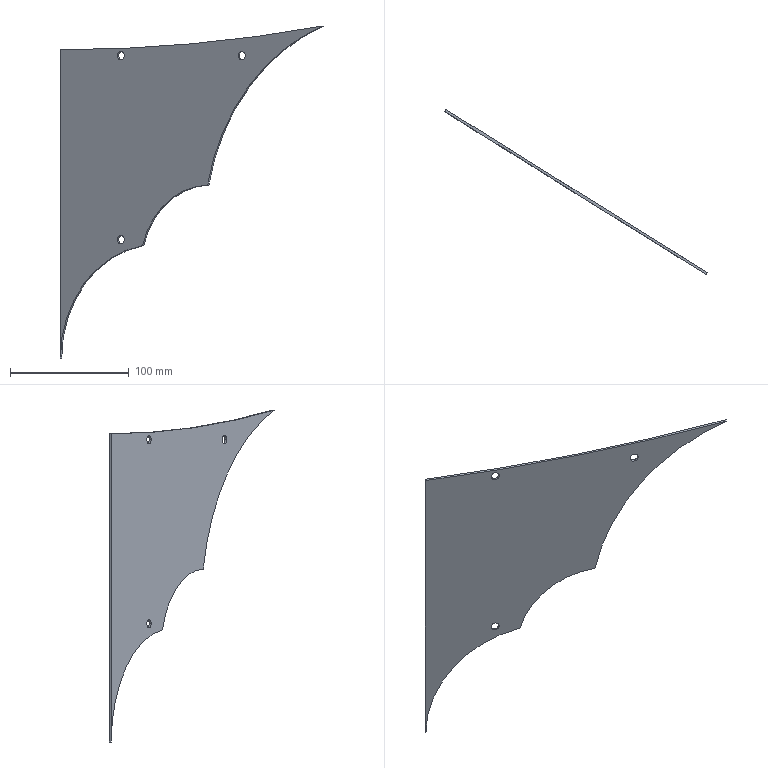Component | SolidWorks | OuterWing-2 | 1 solid | 13 faces | box 221.61 x 139.38 x 279.64 mm | volume 55641 mm3 | cylinder 10 | plane 3 | commonest cylinder face diameters 7 x6 3400 x1 361.12 x1 137.802 x1 191.397 x1
build123d program:
from build123d import *

# Parameters (mm, degrees)
SKETCH1_W           = 260
SKETCH1_H           = 165
BOSS_EXTRUDE1_DEPTH = 2
SKETCH2_R           = 3.5
CUT_EXTRUDE1_DEPTH  = 2
BOSS_EXTRUDE2_DEPTH = 2
CUT_EXTRUDE2_DEPTH  = 2
BOSS_EXTRUDE3_DEPTH = 2


with BuildPart() as part:
    # Sketch1 → Boss-Extrude1 (new body)
    with BuildSketch(Plane.XY):
        with Locations((224.486, -82.5)):
            Rectangle(SKETCH1_W, SKETCH1_H)
    extrude(amount=BOSS_EXTRUDE1_DEPTH)

    # Sketch2 → Cut-Extrude1 (cut)
    with BuildSketch(Plane.XY.offset(2)):
        with Locations((154.486, -160)):
            Circle(SKETCH2_R)
        with Locations((274.486, -160)):
            Circle(SKETCH2_R)
        with Locations((154.486, -5)):
            Circle(SKETCH2_R)
    extrude(amount=-CUT_EXTRUDE1_DEPTH, mode=Mode.SUBTRACT)

    # Sketch3 → Boss-Extrude2 (add)
    with BuildSketch(Plane.XY.offset(2)):
        with BuildLine():
            Line((354.486, -165), (354.486, -185))
            ThreePointArc((354.486, -185), (224.87, -170.007), (94.486, -165))
            Line((94.486, -165), (354.486, -165))
        make_face()
    extrude(amount=-BOSS_EXTRUDE2_DEPTH)

    # Sketch4 → Cut-Extrude2 (cut)
    with BuildSketch(Plane.XY.offset(2)):
        with BuildLine():
            Line((175.984, 0), (354.486, 0))
            Line((354.486, 0), (354.486, -185))
            ThreePointArc((354.486, -185), (280.155, -132.818), (240.63, -51.051))
            ThreePointArc((240.63, -51.051), (199.838, -36.25), (175.984, 0))
        make_face()
    extrude(amount=-CUT_EXTRUDE2_DEPTH, mode=Mode.SUBTRACT)

    # Sketch5 → Boss-Extrude3 (add)
    with BuildSketch(Plane(origin=(0, 0, 0), x_dir=(-1, 0, 0), z_dir=(0, 0, -1))):
        with BuildLine():
            Line((-94.486, 0), (-94.486, 94.639))
            ThreePointArc((-94.486, 94.639), (-117.668, 32.192), (-175.984, 0))
            Line((-175.984, 0), (-94.486, 0))
        make_face()
    extrude(amount=-BOSS_EXTRUDE3_DEPTH)


solid = part.part

# Placed as in the assembly
solid = solid.moved(Location((95.28, 103.927, -37.818), (-90, 31.974, 0)))
STEP:
#1=COLOUR_RGB('',0.7922,0.8196,0.9333);
#2=FILL_AREA_STYLE_COLOUR('',#1);
#3=FILL_AREA_STYLE('',(#2));
#4=SURFACE_STYLE_FILL_AREA(#3);
#5=SURFACE_SIDE_STYLE('',(#4));
#6=SURFACE_STYLE_USAGE(.BOTH.,#5);
#7=PRESENTATION_STYLE_ASSIGNMENT((#6));
#8=CARTESIAN_POINT('',(8.794,0.9439,-1.292));
#9=VERTEX_POINT('',#8);
#10=CARTESIAN_POINT('',(9.027,0.7979,-1.292));
#11=VERTEX_POINT('',#10);
#12=CARTESIAN_POINT('',(8.911,0.8709,-1.292));
#13=DIRECTION('',(0.5295,0.8483,-0.));
#14=DIRECTION('',(0.8483,-0.5295,-0.));
#15=AXIS2_PLACEMENT_3D('',#12,#13,#14);
#16=CIRCLE('',#15,0.1378);
#17=EDGE_CURVE('',#9,#11,#16,.T.);
#18=ORIENTED_EDGE('',*,*,#17,.F.);
#19=CARTESIAN_POINT('',(8.835,1.011,-1.292));
#20=VERTEX_POINT('',#19);
#21=CARTESIAN_POINT('',(8.794,0.9439,-1.292));
#22=DIRECTION('',(0.5295,0.8483,-0.));
#23=VECTOR('',#22,39.37);
#24=LINE('',#21,#23);
#25=EDGE_CURVE('',#9,#20,#24,.T.);
#26=ORIENTED_EDGE('',*,*,#25,.T.);
#27=CARTESIAN_POINT('',(9.069,0.8647,-1.292));
#28=VERTEX_POINT('',#27);
#29=CARTESIAN_POINT('',(8.952,0.9377,-1.292));
#30=DIRECTION('',(0.5295,0.8483,-0.));
#31=DIRECTION('',(0.8483,-0.5295,-0.));
#32=AXIS2_PLACEMENT_3D('',#29,#30,#31);
#33=CIRCLE('',#32,0.1378);
#34=EDGE_CURVE('',#20,#28,#33,.T.);
#35=ORIENTED_EDGE('',*,*,#34,.T.);
#36=CARTESIAN_POINT('',(9.027,0.7979,-1.292));
#37=DIRECTION('',(0.5295,0.8483,-0.));
#38=VECTOR('',#37,39.37);
#39=LINE('',#36,#38);
#40=EDGE_CURVE('',#11,#28,#39,.T.);
#41=ORIENTED_EDGE('',*,*,#40,.F.);
#42=EDGE_LOOP('',(#18,#26,#35,#41));
#43=FACE_OUTER_BOUND('',#42,.T.);
#44=CARTESIAN_POINT('',(8.911,0.8709,-1.292));
#45=DIRECTION('',(0.5295,0.8483,-0.));
#46=DIRECTION('',(0.8483,-0.5295,-0.));
#47=AXIS2_PLACEMENT_3D('',#44,#45,#46);
#48=CYLINDRICAL_SURFACE('',#47,0.1378);
#49=ADVANCED_FACE('',(#43),#48,.F.);
#50=CARTESIAN_POINT('',(12.801,-1.558,4.81));
#51=VERTEX_POINT('',#50);
#52=CARTESIAN_POINT('',(13.035,-1.704,4.81));
#53=VERTEX_POINT('',#52);
#54=CARTESIAN_POINT('',(12.918,-1.631,4.81));
#55=DIRECTION('',(0.5295,0.8483,-0.));
#56=DIRECTION('',(0.8483,-0.5295,-0.));
#57=AXIS2_PLACEMENT_3D('',#54,#55,#56);
#58=CIRCLE('',#57,0.1378);
#59=EDGE_CURVE('',#51,#53,#58,.T.);
#60=ORIENTED_EDGE('',*,*,#59,.F.);
#61=CARTESIAN_POINT('',(12.843,-1.491,4.81));
#62=VERTEX_POINT('',#61);
#63=CARTESIAN_POINT('',(12.801,-1.558,4.81));
#64=DIRECTION('',(0.5295,0.8483,-0.));
#65=VECTOR('',#64,39.37);
#66=LINE('',#63,#65);
#67=EDGE_CURVE('',#51,#62,#66,.T.);
#68=ORIENTED_EDGE('',*,*,#67,.T.);
#69=CARTESIAN_POINT('',(13.077,-1.637,4.81));
#70=VERTEX_POINT('',#69);
#71=CARTESIAN_POINT('',(12.96,-1.564,4.81));
#72=DIRECTION('',(0.5295,0.8483,-0.));
#73=DIRECTION('',(0.8483,-0.5295,-0.));
#74=AXIS2_PLACEMENT_3D('',#71,#72,#73);
#75=CIRCLE('',#74,0.1378);
#76=EDGE_CURVE('',#62,#70,#75,.T.);
#77=ORIENTED_EDGE('',*,*,#76,.T.);
#78=CARTESIAN_POINT('',(13.035,-1.704,4.81));
#79=DIRECTION('',(0.5295,0.8483,-0.));
#80=VECTOR('',#79,39.37);
#81=LINE('',#78,#80);
#82=EDGE_CURVE('',#53,#70,#81,.T.);
#83=ORIENTED_EDGE('',*,*,#82,.F.);
#84=EDGE_LOOP('',(#60,#68,#77,#83));
#85=FACE_OUTER_BOUND('',#84,.T.);
#86=CARTESIAN_POINT('',(12.918,-1.631,4.81));
#87=DIRECTION('',(0.5295,0.8483,-0.));
#88=DIRECTION('',(0.8483,-0.5295,-0.));
#89=AXIS2_PLACEMENT_3D('',#86,#87,#88);
#90=CYLINDRICAL_SURFACE('',#89,0.1378);
#91=ADVANCED_FACE('',(#85),#90,.F.);
#92=CARTESIAN_POINT('',(8.794,0.9439,4.81));
#93=VERTEX_POINT('',#92);
#94=CARTESIAN_POINT('',(9.027,0.7979,4.81));
#95=VERTEX_POINT('',#94);
#96=CARTESIAN_POINT('',(8.911,0.8709,4.81));
#97=DIRECTION('',(0.5295,0.8483,-0.));
#98=DIRECTION('',(0.8483,-0.5295,-0.));
#99=AXIS2_PLACEMENT_3D('',#96,#97,#98);
#100=CIRCLE('',#99,0.1378);
#101=EDGE_CURVE('',#93,#95,#100,.T.);
#102=ORIENTED_EDGE('',*,*,#101,.F.);
#103=CARTESIAN_POINT('',(8.835,1.011,4.81));
#104=VERTEX_POINT('',#103);
#105=CARTESIAN_POINT('',(8.794,0.9439,4.81));
#106=DIRECTION('',(0.5295,0.8483,-0.));
#107=VECTOR('',#106,39.37);
#108=LINE('',#105,#107);
#109=EDGE_CURVE('',#93,#104,#108,.T.);
#110=ORIENTED_EDGE('',*,*,#109,.T.);
#111=CARTESIAN_POINT('',(9.069,0.8647,4.81));
#112=VERTEX_POINT('',#111);
#113=CARTESIAN_POINT('',(8.952,0.9377,4.81));
#114=DIRECTION('',(0.5295,0.8483,-0.));
#115=DIRECTION('',(0.8483,-0.5295,-0.));
#116=AXIS2_PLACEMENT_3D('',#113,#114,#115);
#117=CIRCLE('',#116,0.1378);
#118=EDGE_CURVE('',#104,#112,#117,.T.);
#119=ORIENTED_EDGE('',*,*,#118,.T.);
#120=CARTESIAN_POINT('',(9.027,0.7979,4.81));
#121=DIRECTION('',(0.5295,0.8483,-0.));
#122=VECTOR('',#121,39.37);
#123=LINE('',#120,#122);
#124=EDGE_CURVE('',#95,#112,#123,.T.);
#125=ORIENTED_EDGE('',*,*,#124,.F.);
#126=EDGE_LOOP('',(#102,#110,#119,#125));
#127=FACE_OUTER_BOUND('',#126,.T.);
#128=CARTESIAN_POINT('',(8.911,0.8709,4.81));
#129=DIRECTION('',(0.5295,0.8483,-0.));
#130=DIRECTION('',(0.8483,-0.5295,-0.));
#131=AXIS2_PLACEMENT_3D('',#128,#129,#130);
#132=CYLINDRICAL_SURFACE('',#131,0.1378);
#133=ADVANCED_FACE('',(#127),#132,.F.);
#134=CARTESIAN_POINT('',(6.907,2.122,-5.215));
#135=VERTEX_POINT('',#134);
#136=CARTESIAN_POINT('',(6.907,2.122,5.007));
#137=VERTEX_POINT('',#136);
#138=CARTESIAN_POINT('',(6.907,2.122,-1.489));
#139=DIRECTION('',(0.,-0.,1.));
#140=VECTOR('',#139,39.37);
#141=LINE('',#138,#140);
#142=EDGE_CURVE('',#135,#137,#141,.T.);
#143=ORIENTED_EDGE('',*,*,#142,.T.);
#144=CARTESIAN_POINT('',(6.948,2.189,5.007));
#145=VERTEX_POINT('',#144);
#146=CARTESIAN_POINT('',(6.948,2.189,5.007));
#147=DIRECTION('',(-0.5295,-0.8483,0.));
#148=VECTOR('',#147,39.37);
#149=LINE('',#146,#148);
#150=EDGE_CURVE('',#145,#137,#149,.T.);
#151=ORIENTED_EDGE('',*,*,#150,.F.);
#152=CARTESIAN_POINT('',(6.948,2.189,-5.215));
#153=VERTEX_POINT('',#152);
#154=CARTESIAN_POINT('',(6.948,2.189,-1.489));
#155=DIRECTION('',(0.,-0.,1.));
#156=VECTOR('',#155,39.37);
#157=LINE('',#154,#156);
#158=EDGE_CURVE('',#153,#145,#157,.T.);
#159=ORIENTED_EDGE('',*,*,#158,.F.);
#160=CARTESIAN_POINT('',(6.948,2.189,-5.215));
#161=DIRECTION('',(-0.5295,-0.8483,0.));
#162=VECTOR('',#161,39.37);
#163=LINE('',#160,#162);
#164=EDGE_CURVE('',#153,#135,#163,.T.);
#165=ORIENTED_EDGE('',*,*,#164,.T.);
#166=EDGE_LOOP('',(#143,#151,#159,#165));
#167=FACE_OUTER_BOUND('',#166,.T.);
#168=CARTESIAN_POINT('',(6.948,2.189,-1.489));
#169=DIRECTION('',(0.8483,-0.5295,-0.));
#170=DIRECTION('',(-0.5295,-0.8483,0.));
#171=AXIS2_PLACEMENT_3D('',#168,#169,#170);
#172=PLANE('',#171);
#173=ADVANCED_FACE('',(#167),#172,.F.);
#174=CARTESIAN_POINT('',(11.829,-0.8582,0.521));
#175=VERTEX_POINT('',#174);
#176=CARTESIAN_POINT('',(15.632,-3.232,5.795));
#177=VERTEX_POINT('',#176);
#178=CARTESIAN_POINT('',(17.744,-4.55,-0.8637));
#179=DIRECTION('',(0.5295,0.8483,-0.));
#180=DIRECTION('',(-0.8483,0.5295,0.));
#181=AXIS2_PLACEMENT_3D('',#178,#179,#180);
#182=CIRCLE('',#181,7.109);
#183=EDGE_CURVE('',#175,#177,#182,.T.);
#184=ORIENTED_EDGE('',*,*,#183,.F.);
#185=CARTESIAN_POINT('',(9.67,0.4895,-1.489));
#186=VERTEX_POINT('',#185);
#187=CARTESIAN_POINT('',(11.893,-0.898,-2.191));
#188=DIRECTION('',(0.5295,0.8483,-0.));
#189=DIRECTION('',(-0.8483,0.5295,0.));
#190=AXIS2_PLACEMENT_3D('',#187,#188,#189);
#191=CIRCLE('',#190,2.713);
#192=EDGE_CURVE('',#186,#175,#191,.T.);
#193=ORIENTED_EDGE('',*,*,#192,.F.);
#194=CARTESIAN_POINT('',(10.144,0.1935,-5.215));
#195=DIRECTION('',(0.5295,0.8483,-0.));
#196=DIRECTION('',(0.8483,-0.5295,-0.));
#197=AXIS2_PLACEMENT_3D('',#194,#195,#196);
#198=CIRCLE('',#197,3.768);
#199=EDGE_CURVE('',#153,#186,#198,.T.);
#200=ORIENTED_EDGE('',*,*,#199,.F.);
#201=ORIENTED_EDGE('',*,*,#158,.T.);
#202=CARTESIAN_POINT('',(6.948,2.189,71.936));
#203=DIRECTION('',(-0.5295,-0.8483,0.));
#204=DIRECTION('',(-0.8483,0.5295,0.));
#205=AXIS2_PLACEMENT_3D('',#202,#203,#204);
#206=CIRCLE('',#205,66.929);
#207=EDGE_CURVE('',#145,#177,#206,.T.);
#208=ORIENTED_EDGE('',*,*,#207,.T.);
#209=EDGE_LOOP('',(#184,#193,#200,#201,#208));
#210=FACE_OUTER_BOUND('',#209,.T.);
#211=CARTESIAN_POINT('',(8.952,0.9377,-1.292));
#212=DIRECTION('',(0.5295,0.8483,-0.));
#213=DIRECTION('',(0.8483,-0.5295,-0.));
#214=AXIS2_PLACEMENT_3D('',#211,#212,#213);
#215=CIRCLE('',#214,0.1378);
#216=EDGE_CURVE('',#28,#20,#215,.T.);
#217=ORIENTED_EDGE('',*,*,#216,.F.);
#218=ORIENTED_EDGE('',*,*,#34,.F.);
#219=EDGE_LOOP('',(#217,#218));
#220=FACE_BOUND('',#219,.T.);
#221=CARTESIAN_POINT('',(12.96,-1.564,4.81));
#222=DIRECTION('',(0.5295,0.8483,-0.));
#223=DIRECTION('',(0.8483,-0.5295,-0.));
#224=AXIS2_PLACEMENT_3D('',#221,#222,#223);
#225=CIRCLE('',#224,0.1378);
#226=EDGE_CURVE('',#70,#62,#225,.T.);
#227=ORIENTED_EDGE('',*,*,#226,.F.);
#228=ORIENTED_EDGE('',*,*,#76,.F.);
#229=EDGE_LOOP('',(#227,#228));
#230=FACE_BOUND('',#229,.T.);
#231=CARTESIAN_POINT('',(8.952,0.9377,4.81));
#232=DIRECTION('',(0.5295,0.8483,-0.));
#233=DIRECTION('',(0.8483,-0.5295,-0.));
#234=AXIS2_PLACEMENT_3D('',#231,#232,#233);
#235=CIRCLE('',#234,0.1378);
#236=EDGE_CURVE('',#112,#104,#235,.T.);
#237=ORIENTED_EDGE('',*,*,#236,.F.);
#238=ORIENTED_EDGE('',*,*,#118,.F.);
#239=EDGE_LOOP('',(#237,#238));
#240=FACE_BOUND('',#239,.T.);
#241=CARTESIAN_POINT('',(3.793,4.158,-1.489));
#242=DIRECTION('',(0.5295,0.8483,-0.));
#243=DIRECTION('',(0.8483,-0.5295,-0.));
#244=AXIS2_PLACEMENT_3D('',#241,#242,#243);
#245=PLANE('',#244);
#246=ADVANCED_FACE('',(#210,#220,#230,#240),#245,.T.);
#247=CARTESIAN_POINT('',(8.911,0.8709,-1.292));
#248=DIRECTION('',(0.5295,0.8483,-0.));
#249=DIRECTION('',(0.8483,-0.5295,-0.));
#250=AXIS2_PLACEMENT_3D('',#247,#248,#249);
#251=CIRCLE('',#250,0.1378);
#252=EDGE_CURVE('',#11,#9,#251,.T.);
#253=ORIENTED_EDGE('',*,*,#252,.T.);
#254=ORIENTED_EDGE('',*,*,#17,.T.);
#255=EDGE_LOOP('',(#253,#254));
#256=FACE_BOUND('',#255,.T.);
#257=CARTESIAN_POINT('',(12.918,-1.631,4.81));
#258=DIRECTION('',(0.5295,0.8483,-0.));
#259=DIRECTION('',(0.8483,-0.5295,-0.));
#260=AXIS2_PLACEMENT_3D('',#257,#258,#259);
#261=CIRCLE('',#260,0.1378);
#262=EDGE_CURVE('',#53,#51,#261,.T.);
#263=ORIENTED_EDGE('',*,*,#262,.T.);
#264=ORIENTED_EDGE('',*,*,#59,.T.);
#265=EDGE_LOOP('',(#263,#264));
#266=FACE_BOUND('',#265,.T.);
#267=CARTESIAN_POINT('',(8.911,0.8709,4.81));
#268=DIRECTION('',(0.5295,0.8483,-0.));
#269=DIRECTION('',(0.8483,-0.5295,-0.));
#270=AXIS2_PLACEMENT_3D('',#267,#268,#269);
#271=CIRCLE('',#270,0.1378);
#272=EDGE_CURVE('',#95,#93,#271,.T.);
#273=ORIENTED_EDGE('',*,*,#272,.T.);
#274=ORIENTED_EDGE('',*,*,#101,.T.);
#275=EDGE_LOOP('',(#273,#274));
#276=FACE_BOUND('',#275,.T.);
#277=CARTESIAN_POINT('',(9.629,0.4227,-1.489));
#278=VERTEX_POINT('',#277);
#279=CARTESIAN_POINT('',(11.788,-0.925,0.521));
#280=VERTEX_POINT('',#279);
#281=CARTESIAN_POINT('',(11.851,-0.9648,-2.191));
#282=DIRECTION('',(0.5295,0.8483,-0.));
#283=DIRECTION('',(-0.8483,0.5295,0.));
#284=AXIS2_PLACEMENT_3D('',#281,#282,#283);
#285=CIRCLE('',#284,2.713);
#286=EDGE_CURVE('',#278,#280,#285,.T.);
#287=ORIENTED_EDGE('',*,*,#286,.T.);
#288=CARTESIAN_POINT('',(15.59,-3.299,5.795));
#289=VERTEX_POINT('',#288);
#290=CARTESIAN_POINT('',(17.702,-4.617,-0.8637));
#291=DIRECTION('',(0.5295,0.8483,-0.));
#292=DIRECTION('',(-0.8483,0.5295,0.));
#293=AXIS2_PLACEMENT_3D('',#290,#291,#292);
#294=CIRCLE('',#293,7.109);
#295=EDGE_CURVE('',#280,#289,#294,.T.);
#296=ORIENTED_EDGE('',*,*,#295,.T.);
#297=CARTESIAN_POINT('',(6.907,2.122,71.936));
#298=DIRECTION('',(-0.5295,-0.8483,0.));
#299=DIRECTION('',(-0.8483,0.5295,0.));
#300=AXIS2_PLACEMENT_3D('',#297,#298,#299);
#301=CIRCLE('',#300,66.929);
#302=EDGE_CURVE('',#137,#289,#301,.T.);
#303=ORIENTED_EDGE('',*,*,#302,.F.);
#304=ORIENTED_EDGE('',*,*,#142,.F.);
#305=CARTESIAN_POINT('',(10.103,0.1267,-5.215));
#306=DIRECTION('',(0.5295,0.8483,-0.));
#307=DIRECTION('',(0.8483,-0.5295,-0.));
#308=AXIS2_PLACEMENT_3D('',#305,#306,#307);
#309=CIRCLE('',#308,3.768);
#310=EDGE_CURVE('',#135,#278,#309,.T.);
#311=ORIENTED_EDGE('',*,*,#310,.T.);
#312=EDGE_LOOP('',(#287,#296,#303,#304,#311));
#313=FACE_OUTER_BOUND('',#312,.T.);
#314=CARTESIAN_POINT('',(3.751,4.092,-1.489));
#315=DIRECTION('',(0.5295,0.8483,-0.));
#316=DIRECTION('',(0.8483,-0.5295,-0.));
#317=AXIS2_PLACEMENT_3D('',#314,#315,#316);
#318=PLANE('',#317);
#319=ADVANCED_FACE('',(#256,#266,#276,#313),#318,.F.);
#320=ORIENTED_EDGE('',*,*,#109,.F.);
#321=ORIENTED_EDGE('',*,*,#272,.F.);
#322=ORIENTED_EDGE('',*,*,#124,.T.);
#323=ORIENTED_EDGE('',*,*,#236,.T.);
#324=EDGE_LOOP('',(#320,#321,#322,#323));
#325=FACE_OUTER_BOUND('',#324,.T.);
#326=CARTESIAN_POINT('',(8.911,0.8709,4.81));
#327=DIRECTION('',(0.5295,0.8483,-0.));
#328=DIRECTION('',(0.8483,-0.5295,-0.));
#329=AXIS2_PLACEMENT_3D('',#326,#327,#328);
#330=CYLINDRICAL_SURFACE('',#329,0.1378);
#331=ADVANCED_FACE('',(#325),#330,.F.);
#332=ORIENTED_EDGE('',*,*,#67,.F.);
#333=ORIENTED_EDGE('',*,*,#262,.F.);
#334=ORIENTED_EDGE('',*,*,#82,.T.);
#335=ORIENTED_EDGE('',*,*,#226,.T.);
#336=EDGE_LOOP('',(#332,#333,#334,#335));
#337=FACE_OUTER_BOUND('',#336,.T.);
#338=CARTESIAN_POINT('',(12.918,-1.631,4.81));
#339=DIRECTION('',(0.5295,0.8483,-0.));
#340=DIRECTION('',(0.8483,-0.5295,-0.));
#341=AXIS2_PLACEMENT_3D('',#338,#339,#340);
#342=CYLINDRICAL_SURFACE('',#341,0.1378);
#343=ADVANCED_FACE('',(#337),#342,.F.);
#344=ORIENTED_EDGE('',*,*,#25,.F.);
#345=ORIENTED_EDGE('',*,*,#252,.F.);
#346=ORIENTED_EDGE('',*,*,#40,.T.);
#347=ORIENTED_EDGE('',*,*,#216,.T.);
#348=EDGE_LOOP('',(#344,#345,#346,#347));
#349=FACE_OUTER_BOUND('',#348,.T.);
#350=CARTESIAN_POINT('',(8.911,0.8709,-1.292));
#351=DIRECTION('',(0.5295,0.8483,-0.));
#352=DIRECTION('',(0.8483,-0.5295,-0.));
#353=AXIS2_PLACEMENT_3D('',#350,#351,#352);
#354=CYLINDRICAL_SURFACE('',#353,0.1378);
#355=ADVANCED_FACE('',(#349),#354,.F.);
#356=ORIENTED_EDGE('',*,*,#207,.F.);
#357=ORIENTED_EDGE('',*,*,#150,.T.);
#358=ORIENTED_EDGE('',*,*,#302,.T.);
#359=CARTESIAN_POINT('',(15.59,-3.299,5.795));
#360=DIRECTION('',(0.5295,0.8483,-0.));
#361=VECTOR('',#360,39.37);
#362=LINE('',#359,#361);
#363=EDGE_CURVE('',#289,#177,#362,.T.);
#364=ORIENTED_EDGE('',*,*,#363,.T.);
#365=EDGE_LOOP('',(#356,#357,#358,#364));
#366=FACE_OUTER_BOUND('',#365,.T.);
#367=CARTESIAN_POINT('',(6.907,2.122,71.936));
#368=DIRECTION('',(0.5295,0.8483,-0.));
#369=DIRECTION('',(0.8483,-0.5295,-0.));
#370=AXIS2_PLACEMENT_3D('',#367,#368,#369);
#371=CYLINDRICAL_SURFACE('',#370,66.929);
#372=ADVANCED_FACE('',(#366),#371,.F.);
#373=ORIENTED_EDGE('',*,*,#183,.T.);
#374=ORIENTED_EDGE('',*,*,#363,.F.);
#375=ORIENTED_EDGE('',*,*,#295,.F.);
#376=CARTESIAN_POINT('',(11.788,-0.925,0.521));
#377=DIRECTION('',(0.5295,0.8483,-0.));
#378=VECTOR('',#377,39.37);
#379=LINE('',#376,#378);
#380=EDGE_CURVE('',#280,#175,#379,.T.);
#381=ORIENTED_EDGE('',*,*,#380,.T.);
#382=EDGE_LOOP('',(#373,#374,#375,#381));
#383=FACE_OUTER_BOUND('',#382,.T.);
#384=CARTESIAN_POINT('',(17.702,-4.617,-0.8637));
#385=DIRECTION('',(0.5295,0.8483,-0.));
#386=DIRECTION('',(0.8483,-0.5295,-0.));
#387=AXIS2_PLACEMENT_3D('',#384,#385,#386);
#388=CYLINDRICAL_SURFACE('',#387,7.109);
#389=ADVANCED_FACE('',(#383),#388,.F.);
#390=ORIENTED_EDGE('',*,*,#192,.T.);
#391=ORIENTED_EDGE('',*,*,#380,.F.);
#392=ORIENTED_EDGE('',*,*,#286,.F.);
#393=CARTESIAN_POINT('',(9.629,0.4227,-1.489));
#394=DIRECTION('',(0.5295,0.8483,-0.));
#395=VECTOR('',#394,39.37);
#396=LINE('',#393,#395);
#397=EDGE_CURVE('',#278,#186,#396,.T.);
#398=ORIENTED_EDGE('',*,*,#397,.T.);
#399=EDGE_LOOP('',(#390,#391,#392,#398));
#400=FACE_OUTER_BOUND('',#399,.T.);
#401=CARTESIAN_POINT('',(11.851,-0.9648,-2.191));
#402=DIRECTION('',(0.5295,0.8483,-0.));
#403=DIRECTION('',(0.8483,-0.5295,-0.));
#404=AXIS2_PLACEMENT_3D('',#401,#402,#403);
#405=CYLINDRICAL_SURFACE('',#404,2.713);
#406=ADVANCED_FACE('',(#400),#405,.F.);
#407=ORIENTED_EDGE('',*,*,#310,.F.);
#408=ORIENTED_EDGE('',*,*,#164,.F.);
#409=ORIENTED_EDGE('',*,*,#199,.T.);
#410=ORIENTED_EDGE('',*,*,#397,.F.);
#411=EDGE_LOOP('',(#407,#408,#409,#410));
#412=FACE_OUTER_BOUND('',#411,.T.);
#413=CARTESIAN_POINT('',(10.144,0.1935,-5.215));
#414=DIRECTION('',(-0.5295,-0.8483,0.));
#415=DIRECTION('',(-0.8483,0.5295,0.));
#416=AXIS2_PLACEMENT_3D('',#413,#414,#415);
#417=CYLINDRICAL_SURFACE('',#416,3.768);
#418=ADVANCED_FACE('',(#412),#417,.F.);
#419=CLOSED_SHELL('',(#49,#91,#133,#173,#246,#319,#331,#343,#355,#372,#389,#406,#418));
#420=MANIFOLD_SOLID_BREP('',#419);
#421=STYLED_ITEM('',(#7),#420);
#422=(LENGTH_UNIT()NAMED_UNIT(*)SI_UNIT($,.METRE.));
#423=LENGTH_MEASURE_WITH_UNIT(LENGTH_MEASURE(0.0254),#422);
#424=DIMENSIONAL_EXPONENTS(1.,0.,0.,0.,0.,0.,0.);
#425=(CONVERSION_BASED_UNIT('',#423)LENGTH_UNIT()NAMED_UNIT(#424));
#426=UNCERTAINTY_MEASURE_WITH_UNIT(LENGTH_MEASURE(0.00001),#425,'','');
#427=(NAMED_UNIT(*)PLANE_ANGLE_UNIT()SI_UNIT($,.RADIAN.));
#428=(NAMED_UNIT(*)SI_UNIT($,.STERADIAN.)SOLID_ANGLE_UNIT());
#429=(GEOMETRIC_REPRESENTATION_CONTEXT(3)GLOBAL_UNCERTAINTY_ASSIGNED_CONTEXT((#426))GLOBAL_UNIT_ASSIGNED_CONTEXT((#425,#427,#428))REPRESENTATION_CONTEXT('',''));
#430=MECHANICAL_DESIGN_GEOMETRIC_PRESENTATION_REPRESENTATION('',(#421),#429);
#431=CARTESIAN_POINT('',(0.,0.,0.));
#432=DIRECTION('',(0.,0.,1.));
#433=DIRECTION('',(1.,0.,0.));
#434=AXIS2_PLACEMENT_3D('',#431,#432,#433);
#435=(LENGTH_UNIT()NAMED_UNIT(*)SI_UNIT($,.METRE.));
#436=LENGTH_MEASURE_WITH_UNIT(LENGTH_MEASURE(0.0254),#435);
#437=DIMENSIONAL_EXPONENTS(1.,0.,0.,0.,0.,0.,0.);
#438=(CONVERSION_BASED_UNIT('',#436)LENGTH_UNIT()NAMED_UNIT(#437));
#439=UNCERTAINTY_MEASURE_WITH_UNIT(LENGTH_MEASURE(0.00001),#438,'','');
#440=(NAMED_UNIT(*)PLANE_ANGLE_UNIT()SI_UNIT($,.RADIAN.));
#441=(NAMED_UNIT(*)SI_UNIT($,.STERADIAN.)SOLID_ANGLE_UNIT());
#442=(GEOMETRIC_REPRESENTATION_CONTEXT(3)GLOBAL_UNCERTAINTY_ASSIGNED_CONTEXT((#439))GLOBAL_UNIT_ASSIGNED_CONTEXT((#438,#440,#441))REPRESENTATION_CONTEXT('',''));
#443=ADVANCED_BREP_SHAPE_REPRESENTATION('',(#420,#434),#442);
#444=PRESENTATION_LAYER_ASSIGNMENT('','',(#421));